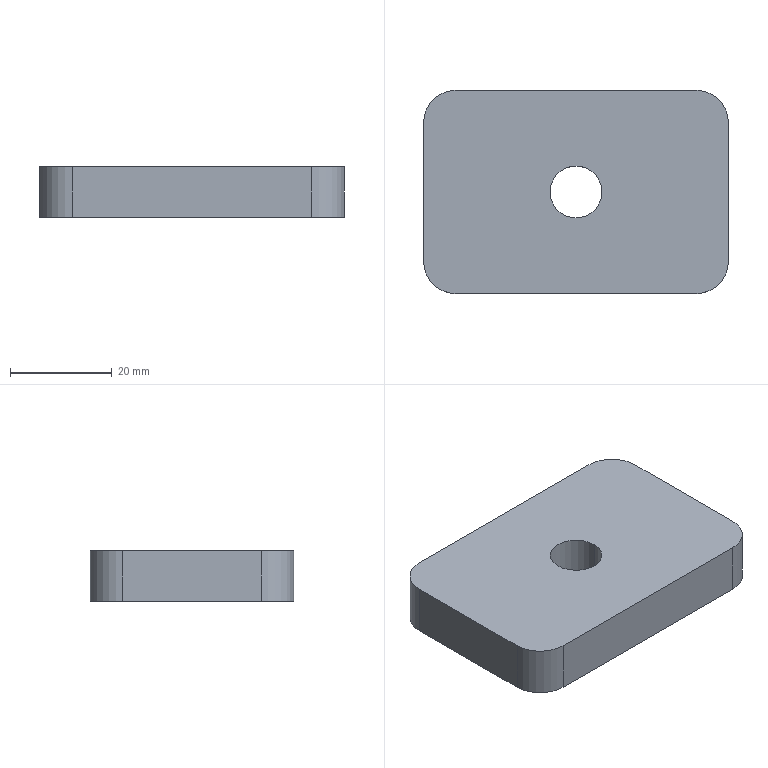Component | SolidWorks | STE21014.03-29-1 | 1 solid | 12 faces | box 60 x 40 x 10 mm | volume 22831 mm3 | cylinder 6 | plane 6 | commonest cylinder face diameters 12.8 x4 10.2 x2 | material Q235
build123d program:
from build123d import *

# Parameters (mm, degrees)
SKETCH1_W              = 40
SKETCH1_H              = 60
BOSS_EXTRUDE1_DEPTH    = 10
FILLET1_R              = 6.4
M12_TAPPED_HOLE1_D     = 10.2
M12_TAPPED_HOLE1_DEPTH = 29.25
M12_TAPPED_HOLE1_TIP   = 3.064


with BuildPart() as part:
    # Sketch1 → Boss-Extrude1 (new body)
    with BuildSketch(Plane(origin=(0, 0, 0), x_dir=(1, 0, 0), z_dir=(0, 1, 0))):
        Rectangle(SKETCH1_W, SKETCH1_H)
    extrude(amount=BOSS_EXTRUDE1_DEPTH)

    # Fillet1
    fillet1_edges = [part.edges().sort_by_distance(p)[0] for p in [
        (-20, 5, -30),
        (20, 5, -30),
        (20, 5, 30),
        (-20, 5, 30),
    ]]
    fillet(fillet1_edges, radius=FILLET1_R)

    # M12 Tapped Hole1
    with Locations(Plane(origin=(0, 10, 0), x_dir=(1, 0, 0), z_dir=(0, 1, 0))):
        with Locations((0, 0)):
            Hole(M12_TAPPED_HOLE1_D / 2, depth=M12_TAPPED_HOLE1_DEPTH)
            with Locations((0, 0, -(M12_TAPPED_HOLE1_DEPTH + M12_TAPPED_HOLE1_TIP / 2))):  # 118° drill point
                Cone(0, M12_TAPPED_HOLE1_D / 2, M12_TAPPED_HOLE1_TIP, mode=Mode.SUBTRACT)


solid = part.part

# Placed as in the assembly
solid = solid.moved(Location((0, 0, 0), (90, -90, 0)))
STEP:
#1=CARTESIAN_POINT('',(-0.2008,-0.,0.3937));
#2=VERTEX_POINT('',#1);
#3=CARTESIAN_POINT('',(0.2008,-0.,0.3937));
#4=VERTEX_POINT('',#3);
#5=CARTESIAN_POINT('',(-0.,-0.,0.3937));
#6=DIRECTION('',(-0.,0.,-1.));
#7=DIRECTION('',(1.,0.,-0.));
#8=AXIS2_PLACEMENT_3D('',#5,#6,#7);
#9=CIRCLE('',#8,0.2008);
#10=EDGE_CURVE('',#2,#4,#9,.T.);
#11=ORIENTED_EDGE('',*,*,#10,.F.);
#12=CARTESIAN_POINT('',(-0.2008,-0.,0.));
#13=VERTEX_POINT('',#12);
#14=CARTESIAN_POINT('',(-0.2008,-0.,0.));
#15=DIRECTION('',(-0.,0.,-1.));
#16=VECTOR('',#15,39.37);
#17=LINE('',#14,#16);
#18=EDGE_CURVE('',#2,#13,#17,.T.);
#19=ORIENTED_EDGE('',*,*,#18,.T.);
#20=CARTESIAN_POINT('',(0.2008,0.,0.));
#21=VERTEX_POINT('',#20);
#22=CARTESIAN_POINT('',(-0.,-0.,0.));
#23=DIRECTION('',(-0.,0.,-1.));
#24=DIRECTION('',(1.,0.,-0.));
#25=AXIS2_PLACEMENT_3D('',#22,#23,#24);
#26=CIRCLE('',#25,0.2008);
#27=EDGE_CURVE('',#13,#21,#26,.T.);
#28=ORIENTED_EDGE('',*,*,#27,.T.);
#29=CARTESIAN_POINT('',(0.2008,0.,0.));
#30=DIRECTION('',(-0.,0.,-1.));
#31=VECTOR('',#30,39.37);
#32=LINE('',#29,#31);
#33=EDGE_CURVE('',#4,#21,#32,.T.);
#34=ORIENTED_EDGE('',*,*,#33,.F.);
#35=EDGE_LOOP('',(#11,#19,#28,#34));
#36=FACE_OUTER_BOUND('',#35,.T.);
#37=CARTESIAN_POINT('',(-0.,-0.,0.));
#38=DIRECTION('',(-0.,0.,-1.));
#39=DIRECTION('',(1.,0.,-0.));
#40=AXIS2_PLACEMENT_3D('',#37,#38,#39);
#41=CYLINDRICAL_SURFACE('',#40,0.2008);
#42=ADVANCED_FACE('',(#36),#41,.F.);
#43=CARTESIAN_POINT('',(-0.9291,0.7874,0.));
#44=VERTEX_POINT('',#43);
#45=CARTESIAN_POINT('',(0.9291,0.7874,0.));
#46=VERTEX_POINT('',#45);
#47=CARTESIAN_POINT('',(1.181,0.7874,0.));
#48=DIRECTION('',(1.,0.,-0.));
#49=VECTOR('',#48,39.37);
#50=LINE('',#47,#49);
#51=EDGE_CURVE('',#44,#46,#50,.T.);
#52=ORIENTED_EDGE('',*,*,#51,.F.);
#53=CARTESIAN_POINT('',(-0.9291,0.7874,0.3937));
#54=VERTEX_POINT('',#53);
#55=CARTESIAN_POINT('',(-0.9291,0.7874,0.));
#56=DIRECTION('',(0.,-0.,1.));
#57=VECTOR('',#56,39.37);
#58=LINE('',#55,#57);
#59=EDGE_CURVE('',#44,#54,#58,.T.);
#60=ORIENTED_EDGE('',*,*,#59,.T.);
#61=CARTESIAN_POINT('',(0.9291,0.7874,0.3937));
#62=VERTEX_POINT('',#61);
#63=CARTESIAN_POINT('',(1.181,0.7874,0.3937));
#64=DIRECTION('',(1.,0.,-0.));
#65=VECTOR('',#64,39.37);
#66=LINE('',#63,#65);
#67=EDGE_CURVE('',#54,#62,#66,.T.);
#68=ORIENTED_EDGE('',*,*,#67,.T.);
#69=CARTESIAN_POINT('',(0.9291,0.7874,0.));
#70=DIRECTION('',(-0.,0.,-1.));
#71=VECTOR('',#70,39.37);
#72=LINE('',#69,#71);
#73=EDGE_CURVE('',#62,#46,#72,.T.);
#74=ORIENTED_EDGE('',*,*,#73,.T.);
#75=EDGE_LOOP('',(#52,#60,#68,#74));
#76=FACE_OUTER_BOUND('',#75,.T.);
#77=CARTESIAN_POINT('',(1.181,0.7874,0.));
#78=DIRECTION('',(0.,-1.,-0.));
#79=DIRECTION('',(-1.,-0.,0.));
#80=AXIS2_PLACEMENT_3D('',#77,#78,#79);
#81=PLANE('',#80);
#82=ADVANCED_FACE('',(#76),#81,.F.);
#83=CARTESIAN_POINT('',(1.181,0.5354,0.3937));
#84=VERTEX_POINT('',#83);
#85=CARTESIAN_POINT('',(1.181,-0.5354,0.3937));
#86=VERTEX_POINT('',#85);
#87=CARTESIAN_POINT('',(1.181,-0.7874,0.3937));
#88=DIRECTION('',(0.,-1.,-0.));
#89=VECTOR('',#88,39.37);
#90=LINE('',#87,#89);
#91=EDGE_CURVE('',#84,#86,#90,.T.);
#92=ORIENTED_EDGE('',*,*,#91,.T.);
#93=CARTESIAN_POINT('',(1.181,-0.5354,0.));
#94=VERTEX_POINT('',#93);
#95=CARTESIAN_POINT('',(1.181,-0.5354,0.));
#96=DIRECTION('',(-0.,0.,-1.));
#97=VECTOR('',#96,39.37);
#98=LINE('',#95,#97);
#99=EDGE_CURVE('',#86,#94,#98,.T.);
#100=ORIENTED_EDGE('',*,*,#99,.T.);
#101=CARTESIAN_POINT('',(1.181,0.5354,0.));
#102=VERTEX_POINT('',#101);
#103=CARTESIAN_POINT('',(1.181,-0.7874,0.));
#104=DIRECTION('',(0.,-1.,-0.));
#105=VECTOR('',#104,39.37);
#106=LINE('',#103,#105);
#107=EDGE_CURVE('',#102,#94,#106,.T.);
#108=ORIENTED_EDGE('',*,*,#107,.F.);
#109=CARTESIAN_POINT('',(1.181,0.5354,0.));
#110=DIRECTION('',(0.,-0.,1.));
#111=VECTOR('',#110,39.37);
#112=LINE('',#109,#111);
#113=EDGE_CURVE('',#102,#84,#112,.T.);
#114=ORIENTED_EDGE('',*,*,#113,.T.);
#115=EDGE_LOOP('',(#92,#100,#108,#114));
#116=FACE_OUTER_BOUND('',#115,.T.);
#117=CARTESIAN_POINT('',(1.181,-0.7874,0.));
#118=DIRECTION('',(-1.,-0.,0.));
#119=DIRECTION('',(-0.,1.,0.));
#120=AXIS2_PLACEMENT_3D('',#117,#118,#119);
#121=PLANE('',#120);
#122=ADVANCED_FACE('',(#116),#121,.F.);
#123=CARTESIAN_POINT('',(0.9291,-0.7874,0.));
#124=VERTEX_POINT('',#123);
#125=CARTESIAN_POINT('',(-0.9291,-0.7874,0.));
#126=VERTEX_POINT('',#125);
#127=CARTESIAN_POINT('',(1.181,-0.7874,0.));
#128=DIRECTION('',(-1.,-0.,0.));
#129=VECTOR('',#128,39.37);
#130=LINE('',#127,#129);
#131=EDGE_CURVE('',#124,#126,#130,.T.);
#132=ORIENTED_EDGE('',*,*,#131,.F.);
#133=CARTESIAN_POINT('',(0.9291,-0.7874,0.3937));
#134=VERTEX_POINT('',#133);
#135=CARTESIAN_POINT('',(0.9291,-0.7874,0.));
#136=DIRECTION('',(0.,-0.,1.));
#137=VECTOR('',#136,39.37);
#138=LINE('',#135,#137);
#139=EDGE_CURVE('',#124,#134,#138,.T.);
#140=ORIENTED_EDGE('',*,*,#139,.T.);
#141=CARTESIAN_POINT('',(-0.9291,-0.7874,0.3937));
#142=VERTEX_POINT('',#141);
#143=CARTESIAN_POINT('',(1.181,-0.7874,0.3937));
#144=DIRECTION('',(-1.,-0.,0.));
#145=VECTOR('',#144,39.37);
#146=LINE('',#143,#145);
#147=EDGE_CURVE('',#134,#142,#146,.T.);
#148=ORIENTED_EDGE('',*,*,#147,.T.);
#149=CARTESIAN_POINT('',(-0.9291,-0.7874,0.));
#150=DIRECTION('',(-0.,0.,-1.));
#151=VECTOR('',#150,39.37);
#152=LINE('',#149,#151);
#153=EDGE_CURVE('',#142,#126,#152,.T.);
#154=ORIENTED_EDGE('',*,*,#153,.T.);
#155=EDGE_LOOP('',(#132,#140,#148,#154));
#156=FACE_OUTER_BOUND('',#155,.T.);
#157=CARTESIAN_POINT('',(1.181,-0.7874,0.));
#158=DIRECTION('',(-0.,1.,0.));
#159=DIRECTION('',(1.,0.,-0.));
#160=AXIS2_PLACEMENT_3D('',#157,#158,#159);
#161=PLANE('',#160);
#162=ADVANCED_FACE('',(#156),#161,.F.);
#163=CARTESIAN_POINT('',(-1.181,-0.5354,0.));
#164=VERTEX_POINT('',#163);
#165=CARTESIAN_POINT('',(-1.181,0.5354,0.));
#166=VERTEX_POINT('',#165);
#167=CARTESIAN_POINT('',(-1.181,-0.7874,0.));
#168=DIRECTION('',(-0.,1.,0.));
#169=VECTOR('',#168,39.37);
#170=LINE('',#167,#169);
#171=EDGE_CURVE('',#164,#166,#170,.T.);
#172=ORIENTED_EDGE('',*,*,#171,.F.);
#173=CARTESIAN_POINT('',(-1.181,-0.5354,0.3937));
#174=VERTEX_POINT('',#173);
#175=CARTESIAN_POINT('',(-1.181,-0.5354,0.));
#176=DIRECTION('',(0.,-0.,1.));
#177=VECTOR('',#176,39.37);
#178=LINE('',#175,#177);
#179=EDGE_CURVE('',#164,#174,#178,.T.);
#180=ORIENTED_EDGE('',*,*,#179,.T.);
#181=CARTESIAN_POINT('',(-1.181,0.5354,0.3937));
#182=VERTEX_POINT('',#181);
#183=CARTESIAN_POINT('',(-1.181,-0.7874,0.3937));
#184=DIRECTION('',(-0.,1.,0.));
#185=VECTOR('',#184,39.37);
#186=LINE('',#183,#185);
#187=EDGE_CURVE('',#174,#182,#186,.T.);
#188=ORIENTED_EDGE('',*,*,#187,.T.);
#189=CARTESIAN_POINT('',(-1.181,0.5354,0.));
#190=DIRECTION('',(-0.,0.,-1.));
#191=VECTOR('',#190,39.37);
#192=LINE('',#189,#191);
#193=EDGE_CURVE('',#182,#166,#192,.T.);
#194=ORIENTED_EDGE('',*,*,#193,.T.);
#195=EDGE_LOOP('',(#172,#180,#188,#194));
#196=FACE_OUTER_BOUND('',#195,.T.);
#197=CARTESIAN_POINT('',(-1.181,-0.7874,0.));
#198=DIRECTION('',(1.,0.,-0.));
#199=DIRECTION('',(0.,-1.,-0.));
#200=AXIS2_PLACEMENT_3D('',#197,#198,#199);
#201=PLANE('',#200);
#202=ADVANCED_FACE('',(#196),#201,.F.);
#203=CARTESIAN_POINT('',(-0.,-0.,0.));
#204=DIRECTION('',(-0.,0.,-1.));
#205=DIRECTION('',(1.,0.,-0.));
#206=AXIS2_PLACEMENT_3D('',#203,#204,#205);
#207=CIRCLE('',#206,0.2008);
#208=EDGE_CURVE('',#21,#13,#207,.T.);
#209=ORIENTED_EDGE('',*,*,#208,.F.);
#210=ORIENTED_EDGE('',*,*,#27,.F.);
#211=EDGE_LOOP('',(#209,#210));
#212=FACE_BOUND('',#211,.T.);
#213=ORIENTED_EDGE('',*,*,#107,.T.);
#214=CARTESIAN_POINT('',(0.9291,-0.5354,0.));
#215=DIRECTION('',(-0.,0.,-1.));
#216=DIRECTION('',(1.,0.,-0.));
#217=AXIS2_PLACEMENT_3D('',#214,#215,#216);
#218=CIRCLE('',#217,0.252);
#219=EDGE_CURVE('',#94,#124,#218,.T.);
#220=ORIENTED_EDGE('',*,*,#219,.T.);
#221=ORIENTED_EDGE('',*,*,#131,.T.);
#222=CARTESIAN_POINT('',(-0.9291,-0.5354,0.));
#223=DIRECTION('',(-0.,0.,-1.));
#224=DIRECTION('',(1.,0.,-0.));
#225=AXIS2_PLACEMENT_3D('',#222,#223,#224);
#226=CIRCLE('',#225,0.252);
#227=EDGE_CURVE('',#126,#164,#226,.T.);
#228=ORIENTED_EDGE('',*,*,#227,.T.);
#229=ORIENTED_EDGE('',*,*,#171,.T.);
#230=CARTESIAN_POINT('',(-0.9291,0.5354,0.));
#231=DIRECTION('',(-0.,0.,-1.));
#232=DIRECTION('',(1.,0.,-0.));
#233=AXIS2_PLACEMENT_3D('',#230,#231,#232);
#234=CIRCLE('',#233,0.252);
#235=EDGE_CURVE('',#166,#44,#234,.T.);
#236=ORIENTED_EDGE('',*,*,#235,.T.);
#237=ORIENTED_EDGE('',*,*,#51,.T.);
#238=CARTESIAN_POINT('',(0.9291,0.5354,0.));
#239=DIRECTION('',(-0.,0.,-1.));
#240=DIRECTION('',(1.,0.,-0.));
#241=AXIS2_PLACEMENT_3D('',#238,#239,#240);
#242=CIRCLE('',#241,0.252);
#243=EDGE_CURVE('',#46,#102,#242,.T.);
#244=ORIENTED_EDGE('',*,*,#243,.T.);
#245=EDGE_LOOP('',(#213,#220,#221,#228,#229,#236,#237,#244));
#246=FACE_OUTER_BOUND('',#245,.T.);
#247=CARTESIAN_POINT('',(-0.,-0.,0.));
#248=DIRECTION('',(-0.,0.,-1.));
#249=DIRECTION('',(1.,0.,-0.));
#250=AXIS2_PLACEMENT_3D('',#247,#248,#249);
#251=PLANE('',#250);
#252=ADVANCED_FACE('',(#212,#246),#251,.T.);
#253=CARTESIAN_POINT('',(-0.,-0.,0.3937));
#254=DIRECTION('',(-0.,0.,-1.));
#255=DIRECTION('',(1.,0.,-0.));
#256=AXIS2_PLACEMENT_3D('',#253,#254,#255);
#257=CIRCLE('',#256,0.2008);
#258=EDGE_CURVE('',#4,#2,#257,.T.);
#259=ORIENTED_EDGE('',*,*,#258,.T.);
#260=ORIENTED_EDGE('',*,*,#10,.T.);
#261=EDGE_LOOP('',(#259,#260));
#262=FACE_BOUND('',#261,.T.);
#263=ORIENTED_EDGE('',*,*,#147,.F.);
#264=CARTESIAN_POINT('',(0.9291,-0.5354,0.3937));
#265=DIRECTION('',(0.,-0.,1.));
#266=DIRECTION('',(1.,0.,-0.));
#267=AXIS2_PLACEMENT_3D('',#264,#265,#266);
#268=CIRCLE('',#267,0.252);
#269=EDGE_CURVE('',#134,#86,#268,.T.);
#270=ORIENTED_EDGE('',*,*,#269,.T.);
#271=ORIENTED_EDGE('',*,*,#91,.F.);
#272=CARTESIAN_POINT('',(0.9291,0.5354,0.3937));
#273=DIRECTION('',(0.,-0.,1.));
#274=DIRECTION('',(1.,0.,-0.));
#275=AXIS2_PLACEMENT_3D('',#272,#273,#274);
#276=CIRCLE('',#275,0.252);
#277=EDGE_CURVE('',#84,#62,#276,.T.);
#278=ORIENTED_EDGE('',*,*,#277,.T.);
#279=ORIENTED_EDGE('',*,*,#67,.F.);
#280=CARTESIAN_POINT('',(-0.9291,0.5354,0.3937));
#281=DIRECTION('',(0.,-0.,1.));
#282=DIRECTION('',(1.,0.,-0.));
#283=AXIS2_PLACEMENT_3D('',#280,#281,#282);
#284=CIRCLE('',#283,0.252);
#285=EDGE_CURVE('',#54,#182,#284,.T.);
#286=ORIENTED_EDGE('',*,*,#285,.T.);
#287=ORIENTED_EDGE('',*,*,#187,.F.);
#288=CARTESIAN_POINT('',(-0.9291,-0.5354,0.3937));
#289=DIRECTION('',(0.,-0.,1.));
#290=DIRECTION('',(1.,0.,-0.));
#291=AXIS2_PLACEMENT_3D('',#288,#289,#290);
#292=CIRCLE('',#291,0.252);
#293=EDGE_CURVE('',#174,#142,#292,.T.);
#294=ORIENTED_EDGE('',*,*,#293,.T.);
#295=EDGE_LOOP('',(#263,#270,#271,#278,#279,#286,#287,#294));
#296=FACE_OUTER_BOUND('',#295,.T.);
#297=CARTESIAN_POINT('',(-0.,-0.,0.3937));
#298=DIRECTION('',(-0.,0.,-1.));
#299=DIRECTION('',(1.,0.,-0.));
#300=AXIS2_PLACEMENT_3D('',#297,#298,#299);
#301=PLANE('',#300);
#302=ADVANCED_FACE('',(#262,#296),#301,.F.);
#303=ORIENTED_EDGE('',*,*,#219,.F.);
#304=ORIENTED_EDGE('',*,*,#99,.F.);
#305=ORIENTED_EDGE('',*,*,#269,.F.);
#306=ORIENTED_EDGE('',*,*,#139,.F.);
#307=EDGE_LOOP('',(#303,#304,#305,#306));
#308=FACE_OUTER_BOUND('',#307,.T.);
#309=CARTESIAN_POINT('',(0.9291,-0.5354,0.));
#310=DIRECTION('',(0.,-0.,1.));
#311=DIRECTION('',(-1.,-0.,0.));
#312=AXIS2_PLACEMENT_3D('',#309,#310,#311);
#313=CYLINDRICAL_SURFACE('',#312,0.252);
#314=ADVANCED_FACE('',(#308),#313,.T.);
#315=ORIENTED_EDGE('',*,*,#227,.F.);
#316=ORIENTED_EDGE('',*,*,#153,.F.);
#317=ORIENTED_EDGE('',*,*,#293,.F.);
#318=ORIENTED_EDGE('',*,*,#179,.F.);
#319=EDGE_LOOP('',(#315,#316,#317,#318));
#320=FACE_OUTER_BOUND('',#319,.T.);
#321=CARTESIAN_POINT('',(-0.9291,-0.5354,0.));
#322=DIRECTION('',(0.,-0.,1.));
#323=DIRECTION('',(-1.,-0.,0.));
#324=AXIS2_PLACEMENT_3D('',#321,#322,#323);
#325=CYLINDRICAL_SURFACE('',#324,0.252);
#326=ADVANCED_FACE('',(#320),#325,.T.);
#327=ORIENTED_EDGE('',*,*,#235,.F.);
#328=ORIENTED_EDGE('',*,*,#193,.F.);
#329=ORIENTED_EDGE('',*,*,#285,.F.);
#330=ORIENTED_EDGE('',*,*,#59,.F.);
#331=EDGE_LOOP('',(#327,#328,#329,#330));
#332=FACE_OUTER_BOUND('',#331,.T.);
#333=CARTESIAN_POINT('',(-0.9291,0.5354,0.));
#334=DIRECTION('',(0.,-0.,1.));
#335=DIRECTION('',(-1.,-0.,0.));
#336=AXIS2_PLACEMENT_3D('',#333,#334,#335);
#337=CYLINDRICAL_SURFACE('',#336,0.252);
#338=ADVANCED_FACE('',(#332),#337,.T.);
#339=ORIENTED_EDGE('',*,*,#243,.F.);
#340=ORIENTED_EDGE('',*,*,#73,.F.);
#341=ORIENTED_EDGE('',*,*,#277,.F.);
#342=ORIENTED_EDGE('',*,*,#113,.F.);
#343=EDGE_LOOP('',(#339,#340,#341,#342));
#344=FACE_OUTER_BOUND('',#343,.T.);
#345=CARTESIAN_POINT('',(0.9291,0.5354,0.));
#346=DIRECTION('',(0.,-0.,1.));
#347=DIRECTION('',(-1.,-0.,0.));
#348=AXIS2_PLACEMENT_3D('',#345,#346,#347);
#349=CYLINDRICAL_SURFACE('',#348,0.252);
#350=ADVANCED_FACE('',(#344),#349,.T.);
#351=ORIENTED_EDGE('',*,*,#18,.F.);
#352=ORIENTED_EDGE('',*,*,#258,.F.);
#353=ORIENTED_EDGE('',*,*,#33,.T.);
#354=ORIENTED_EDGE('',*,*,#208,.T.);
#355=EDGE_LOOP('',(#351,#352,#353,#354));
#356=FACE_OUTER_BOUND('',#355,.T.);
#357=CARTESIAN_POINT('',(-0.,-0.,0.));
#358=DIRECTION('',(-0.,0.,-1.));
#359=DIRECTION('',(1.,0.,-0.));
#360=AXIS2_PLACEMENT_3D('',#357,#358,#359);
#361=CYLINDRICAL_SURFACE('',#360,0.2008);
#362=ADVANCED_FACE('',(#356),#361,.F.);
#363=CLOSED_SHELL('',(#42,#82,#122,#162,#202,#252,#302,#314,#326,#338,#350,#362));
#364=MANIFOLD_SOLID_BREP('',#363);
#365=CARTESIAN_POINT('',(0.,0.,0.));
#366=DIRECTION('',(0.,0.,1.));
#367=DIRECTION('',(1.,0.,0.));
#368=AXIS2_PLACEMENT_3D('',#365,#366,#367);
#369=(LENGTH_UNIT()NAMED_UNIT(*)SI_UNIT($,.METRE.));
#370=LENGTH_MEASURE_WITH_UNIT(LENGTH_MEASURE(0.0254),#369);
#371=DIMENSIONAL_EXPONENTS(1.,0.,0.,0.,0.,0.,0.);
#372=(CONVERSION_BASED_UNIT('',#370)LENGTH_UNIT()NAMED_UNIT(#371));
#373=UNCERTAINTY_MEASURE_WITH_UNIT(LENGTH_MEASURE(0.00001),#372,'','');
#374=(NAMED_UNIT(*)PLANE_ANGLE_UNIT()SI_UNIT($,.RADIAN.));
#375=(NAMED_UNIT(*)SI_UNIT($,.STERADIAN.)SOLID_ANGLE_UNIT());
#376=(GEOMETRIC_REPRESENTATION_CONTEXT(3)GLOBAL_UNCERTAINTY_ASSIGNED_CONTEXT((#373))GLOBAL_UNIT_ASSIGNED_CONTEXT((#372,#374,#375))REPRESENTATION_CONTEXT('',''));
#377=ADVANCED_BREP_SHAPE_REPRESENTATION('',(#364,#368),#376);
#378=COLOUR_RGB('',0.7922,0.8196,0.9333);
#379=FILL_AREA_STYLE_COLOUR('',#378);
#380=FILL_AREA_STYLE('',(#379));
#381=SURFACE_STYLE_FILL_AREA(#380);
#382=SURFACE_SIDE_STYLE('',(#381));
#383=SURFACE_STYLE_USAGE(.BOTH.,#382);
#384=PRESENTATION_STYLE_ASSIGNMENT((#383));
#385=STYLED_ITEM('',(#384),#364);
#386=(LENGTH_UNIT()NAMED_UNIT(*)SI_UNIT($,.METRE.));
#387=LENGTH_MEASURE_WITH_UNIT(LENGTH_MEASURE(0.0254),#386);
#388=DIMENSIONAL_EXPONENTS(1.,0.,0.,0.,0.,0.,0.);
#389=(CONVERSION_BASED_UNIT('',#387)LENGTH_UNIT()NAMED_UNIT(#388));
#390=UNCERTAINTY_MEASURE_WITH_UNIT(LENGTH_MEASURE(0.00001),#389,'','');
#391=(NAMED_UNIT(*)PLANE_ANGLE_UNIT()SI_UNIT($,.RADIAN.));
#392=(NAMED_UNIT(*)SI_UNIT($,.STERADIAN.)SOLID_ANGLE_UNIT());
#393=(GEOMETRIC_REPRESENTATION_CONTEXT(3)GLOBAL_UNCERTAINTY_ASSIGNED_CONTEXT((#390))GLOBAL_UNIT_ASSIGNED_CONTEXT((#389,#391,#392))REPRESENTATION_CONTEXT('',''));
#394=MECHANICAL_DESIGN_GEOMETRIC_PRESENTATION_REPRESENTATION('',(#385),#393);
#395=PRESENTATION_LAYER_ASSIGNMENT('','',(#385));